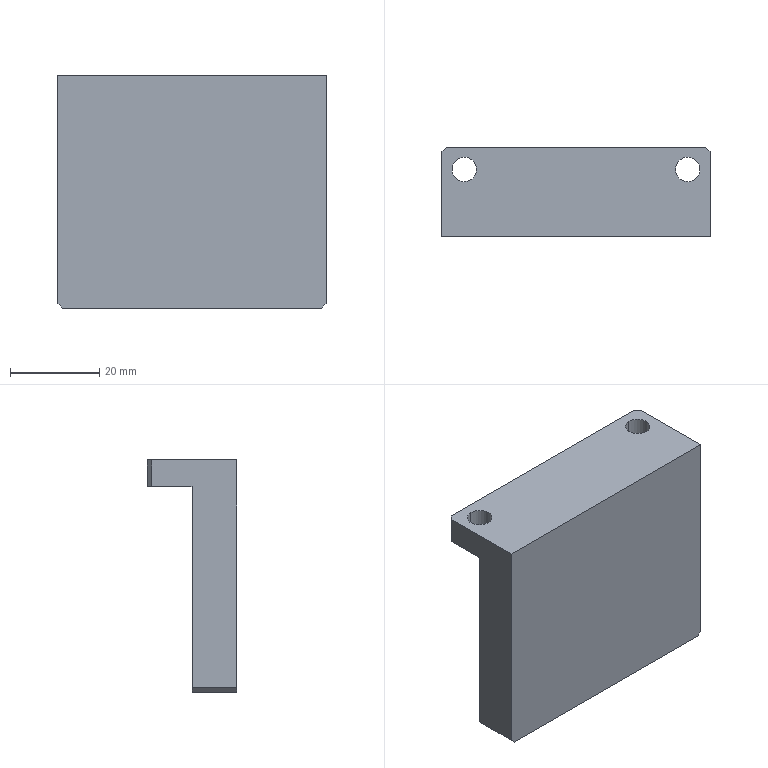CAM job | Mastercam | mm | 12 operations | part box 60 x 20 x 52
1. Facing | 24 - 100 平铣刀
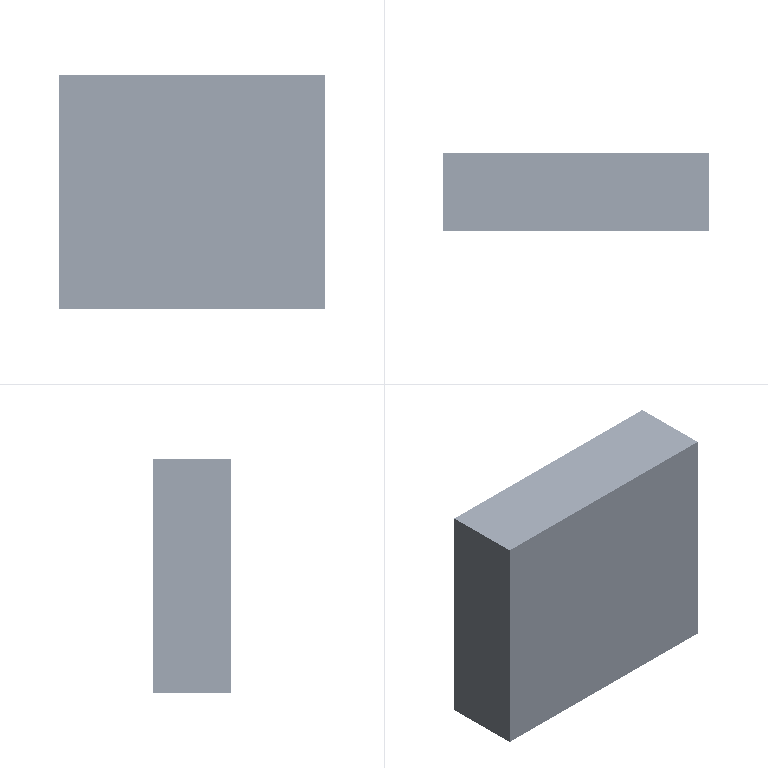2. 2D High Speed (2D Dynamic Mill) | 12 - 12 平铣刀
3. Contour (2D) | 12 - 12 平铣刀
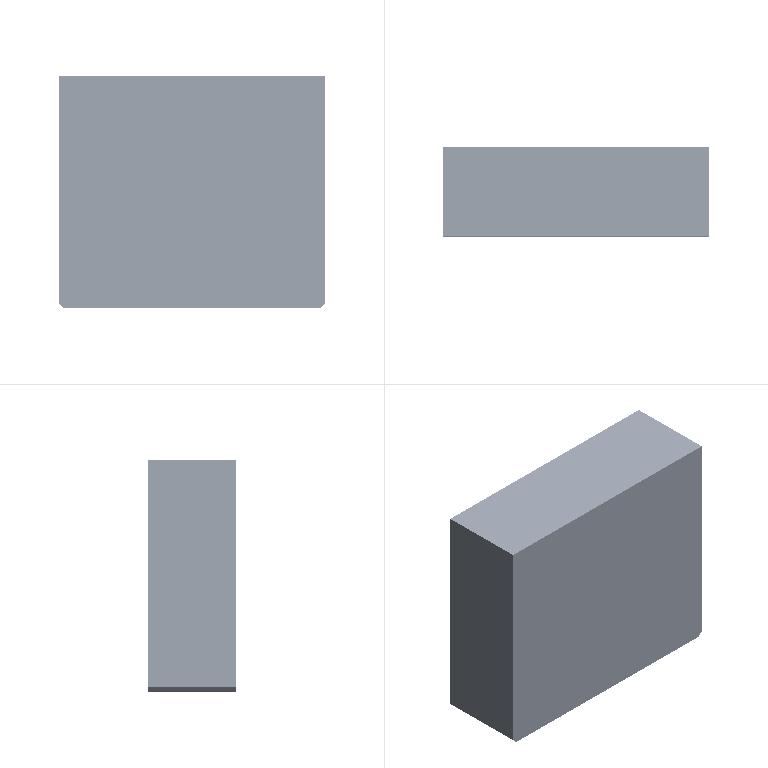4. Contour (2D chamfer) | 7 - 4 倒角刀
5. Facing | 24 - 100 平铣刀
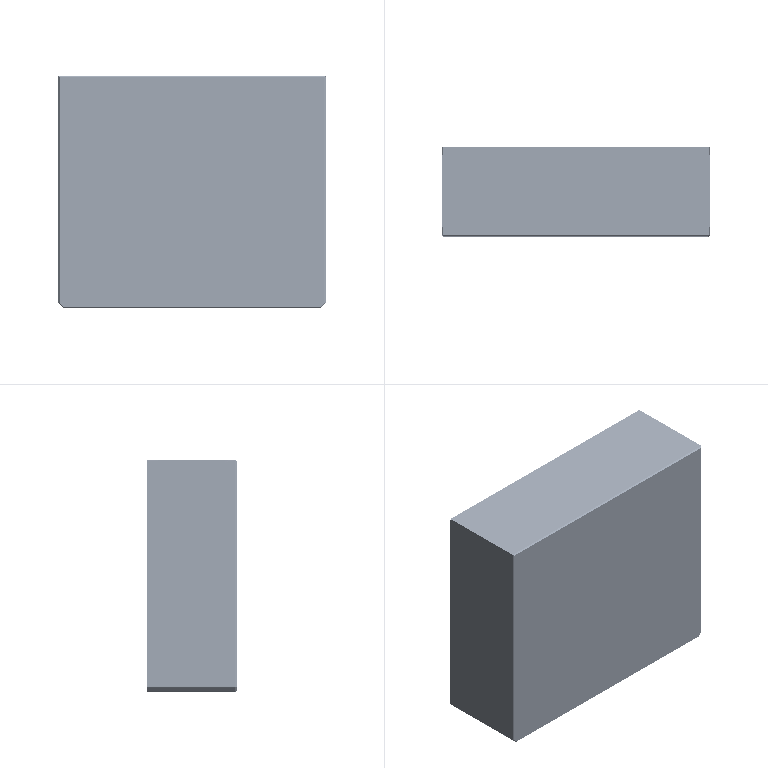6. Contour (Ramp) | 24 - 100 平铣刀
7. Contour (2D) | 12 - 12 平铣刀
8. Contour (2D chamfer) | 7 - 4 倒角刀
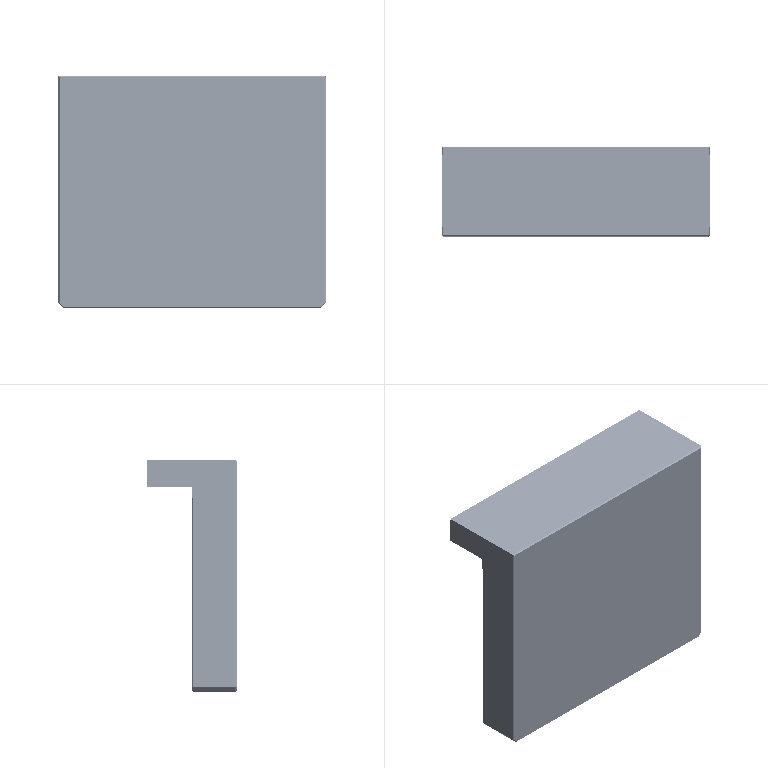9. Contour (2D chamfer) | 7 - 4 倒角刀
10. Contour (2D chamfer) | 7 - 4 倒角刀
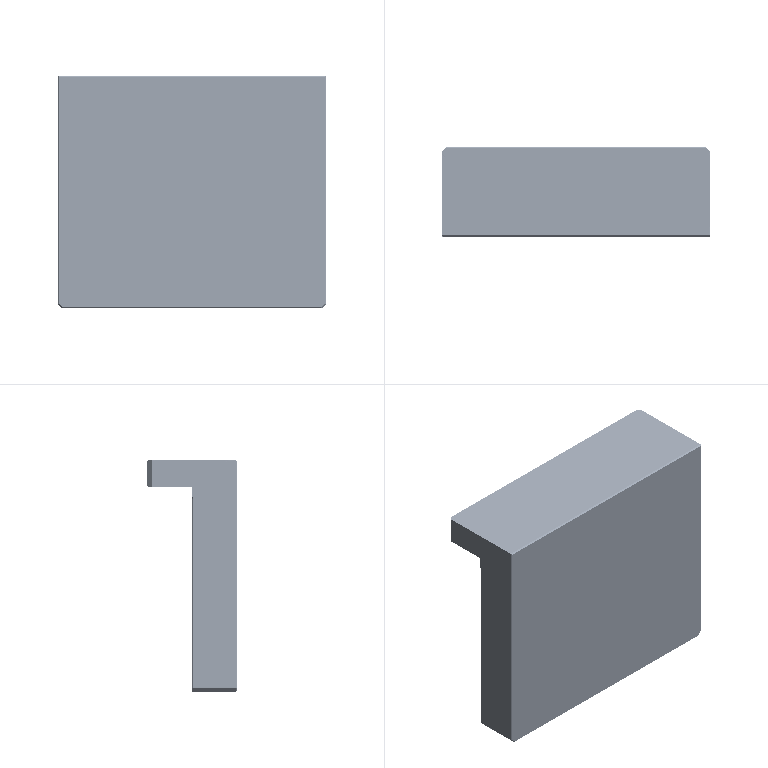11. Drill/Counterbore | 7 - 4 倒角刀
12. Drill/Counterbore | 7 - 4 倒角刀